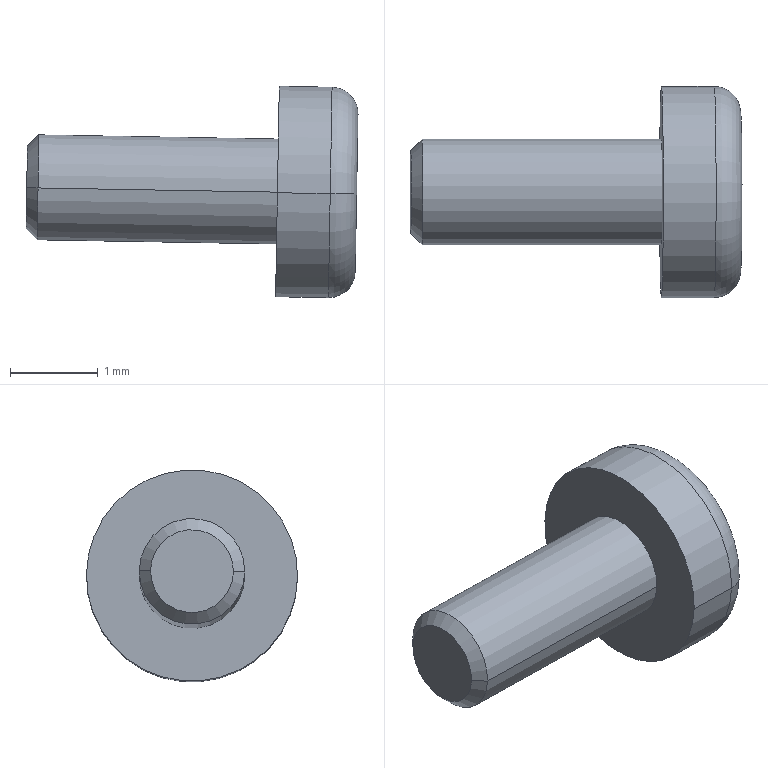Component | SolidWorks | 00-VacuumSuctionCupAssembly-1_06-M4PhillipsScrew-3 | 1 solid | 28 faces | box 3.77 x 2.4 x 2.41 mm | volume 7 mm3 | plane 16 | cylinder 8 | torus 2 | cone 2 | commonest cylinder face diameters 0.42 x4 1.2 x2 2.4 x2
STEP:
#1=CARTESIAN_POINT('',(2.87,5.778,1.592));
#2=VERTEX_POINT('',#1);
#3=CARTESIAN_POINT('',(2.87,5.873,1.594));
#4=VERTEX_POINT('',#3);
#5=CARTESIAN_POINT('',(2.87,5.826,1.593));
#6=DIRECTION('',(-0.9998,0.,0.01745));
#7=DIRECTION('',(0.0001976,0.9999,0.01132));
#8=AXIS2_PLACEMENT_3D('',#5,#6,#7);
#9=CIRCLE('',#8,0.04724);
#10=EDGE_CURVE('',#2,#4,#9,.T.);
#11=ORIENTED_EDGE('',*,*,#10,.F.);
#12=CARTESIAN_POINT('',(2.882,5.79,1.592));
#13=VERTEX_POINT('',#12);
#14=CARTESIAN_POINT('',(2.87,5.79,1.593));
#15=DIRECTION('',(0.01745,-0.01132,0.9998));
#16=DIRECTION('',(0.9998,0.,-0.01745));
#17=AXIS2_PLACEMENT_3D('',#14,#15,#16);
#18=CIRCLE('',#17,0.01181);
#19=EDGE_CURVE('',#2,#13,#18,.T.);
#20=ORIENTED_EDGE('',*,*,#19,.T.);
#21=CARTESIAN_POINT('',(2.882,5.861,1.593));
#22=VERTEX_POINT('',#21);
#23=CARTESIAN_POINT('',(2.882,5.826,1.593));
#24=DIRECTION('',(0.9998,-0.,-0.01745));
#25=DIRECTION('',(0.0001976,0.9999,0.01132));
#26=AXIS2_PLACEMENT_3D('',#23,#24,#25);
#27=CIRCLE('',#26,0.03543);
#28=EDGE_CURVE('',#22,#13,#27,.T.);
#29=ORIENTED_EDGE('',*,*,#28,.F.);
#30=CARTESIAN_POINT('',(2.87,5.861,1.593));
#31=DIRECTION('',(-0.01745,0.01132,-0.9998));
#32=DIRECTION('',(-0.9998,0.,0.01745));
#33=AXIS2_PLACEMENT_3D('',#30,#31,#32);
#34=CIRCLE('',#33,0.01181);
#35=EDGE_CURVE('',#4,#22,#34,.T.);
#36=ORIENTED_EDGE('',*,*,#35,.F.);
#37=EDGE_LOOP('',(#11,#20,#29,#36));
#38=FACE_OUTER_BOUND('',#37,.T.);
#39=CARTESIAN_POINT('',(2.87,5.826,1.593));
#40=DIRECTION('',(0.9998,-0.,-0.01745));
#41=DIRECTION('',(0.0001976,0.9999,0.01132));
#42=AXIS2_PLACEMENT_3D('',#39,#40,#41);
#43=TOROIDAL_SURFACE('',#42,0.03543,0.01181);
#44=ADVANCED_FACE('',(#38),#43,.T.);
#45=CARTESIAN_POINT('',(2.734,5.807,1.595));
#46=VERTEX_POINT('',#45);
#47=CARTESIAN_POINT('',(2.734,5.844,1.596));
#48=VERTEX_POINT('',#47);
#49=CARTESIAN_POINT('',(2.734,5.826,1.595));
#50=DIRECTION('',(-0.9998,0.,0.01745));
#51=DIRECTION('',(-0.0001976,-0.9999,-0.01132));
#52=AXIS2_PLACEMENT_3D('',#49,#50,#51);
#53=CIRCLE('',#52,0.01855);
#54=EDGE_CURVE('',#46,#48,#53,.T.);
#55=ORIENTED_EDGE('',*,*,#54,.F.);
#56=CARTESIAN_POINT('',(2.739,5.802,1.595));
#57=VERTEX_POINT('',#56);
#58=CARTESIAN_POINT('',(2.734,5.807,1.595));
#59=DIRECTION('',(0.7069,-0.7071,-0.02034));
#60=VECTOR('',#59,39.37);
#61=LINE('',#58,#60);
#62=EDGE_CURVE('',#46,#57,#61,.T.);
#63=ORIENTED_EDGE('',*,*,#62,.T.);
#64=CARTESIAN_POINT('',(2.739,5.849,1.596));
#65=VERTEX_POINT('',#64);
#66=CARTESIAN_POINT('',(2.739,5.826,1.595));
#67=DIRECTION('',(0.9998,-0.,-0.01745));
#68=DIRECTION('',(-0.0001976,-0.9999,-0.01132));
#69=AXIS2_PLACEMENT_3D('',#66,#67,#68);
#70=CIRCLE('',#69,0.02362);
#71=EDGE_CURVE('',#65,#57,#70,.T.);
#72=ORIENTED_EDGE('',*,*,#71,.F.);
#73=CARTESIAN_POINT('',(2.734,5.844,1.596));
#74=DIRECTION('',(0.7071,0.7071,-0.004337));
#75=VECTOR('',#74,39.37);
#76=LINE('',#73,#75);
#77=EDGE_CURVE('',#48,#65,#76,.T.);
#78=ORIENTED_EDGE('',*,*,#77,.F.);
#79=EDGE_LOOP('',(#55,#63,#72,#78));
#80=FACE_OUTER_BOUND('',#79,.T.);
#81=CARTESIAN_POINT('',(2.734,5.826,1.595));
#82=DIRECTION('',(0.9998,-0.,-0.01745));
#83=DIRECTION('',(0.0001976,0.9999,0.01132));
#84=AXIS2_PLACEMENT_3D('',#81,#82,#83);
#85=CONICAL_SURFACE('',#84,0.01855,0.7854);
#86=ADVANCED_FACE('',(#80),#85,.T.);
#87=ORIENTED_EDGE('',*,*,#71,.T.);
#88=CARTESIAN_POINT('',(2.846,5.802,1.593));
#89=VERTEX_POINT('',#88);
#90=CARTESIAN_POINT('',(2.734,5.802,1.595));
#91=DIRECTION('',(0.9998,-0.,-0.01745));
#92=VECTOR('',#91,39.37);
#93=LINE('',#90,#92);
#94=EDGE_CURVE('',#57,#89,#93,.T.);
#95=ORIENTED_EDGE('',*,*,#94,.T.);
#96=CARTESIAN_POINT('',(2.846,5.849,1.594));
#97=VERTEX_POINT('',#96);
#98=CARTESIAN_POINT('',(2.846,5.826,1.593));
#99=DIRECTION('',(-0.9998,0.,0.01745));
#100=DIRECTION('',(-0.0001976,-0.9999,-0.01132));
#101=AXIS2_PLACEMENT_3D('',#98,#99,#100);
#102=CIRCLE('',#101,0.02362);
#103=EDGE_CURVE('',#89,#97,#102,.T.);
#104=ORIENTED_EDGE('',*,*,#103,.T.);
#105=CARTESIAN_POINT('',(2.734,5.849,1.596));
#106=DIRECTION('',(0.9998,-0.,-0.01745));
#107=VECTOR('',#106,39.37);
#108=LINE('',#105,#107);
#109=EDGE_CURVE('',#65,#97,#108,.T.);
#110=ORIENTED_EDGE('',*,*,#109,.F.);
#111=EDGE_LOOP('',(#87,#95,#104,#110));
#112=FACE_OUTER_BOUND('',#111,.T.);
#113=CARTESIAN_POINT('',(2.734,5.826,1.595));
#114=DIRECTION('',(0.9998,-0.,-0.01745));
#115=DIRECTION('',(0.0001976,0.9999,0.01132));
#116=AXIS2_PLACEMENT_3D('',#113,#114,#115);
#117=CYLINDRICAL_SURFACE('',#116,0.02362);
#118=ADVANCED_FACE('',(#112),#117,.T.);
#119=ORIENTED_EDGE('',*,*,#10,.T.);
#120=CARTESIAN_POINT('',(2.846,5.873,1.594));
#121=VERTEX_POINT('',#120);
#122=CARTESIAN_POINT('',(2.882,5.873,1.593));
#123=DIRECTION('',(-0.9998,0.,0.01745));
#124=VECTOR('',#123,39.37);
#125=LINE('',#122,#124);
#126=EDGE_CURVE('',#4,#121,#125,.T.);
#127=ORIENTED_EDGE('',*,*,#126,.T.);
#128=CARTESIAN_POINT('',(2.846,5.778,1.593));
#129=VERTEX_POINT('',#128);
#130=CARTESIAN_POINT('',(2.846,5.826,1.593));
#131=DIRECTION('',(-0.9998,0.,0.01745));
#132=DIRECTION('',(-0.0001976,-0.9999,-0.01132));
#133=AXIS2_PLACEMENT_3D('',#130,#131,#132);
#134=CIRCLE('',#133,0.04724);
#135=EDGE_CURVE('',#129,#121,#134,.T.);
#136=ORIENTED_EDGE('',*,*,#135,.F.);
#137=CARTESIAN_POINT('',(2.882,5.778,1.592));
#138=DIRECTION('',(-0.9998,0.,0.01745));
#139=VECTOR('',#138,39.37);
#140=LINE('',#137,#139);
#141=EDGE_CURVE('',#2,#129,#140,.T.);
#142=ORIENTED_EDGE('',*,*,#141,.F.);
#143=EDGE_LOOP('',(#119,#127,#136,#142));
#144=FACE_OUTER_BOUND('',#143,.T.);
#145=CARTESIAN_POINT('',(2.882,5.826,1.593));
#146=DIRECTION('',(-0.9998,0.,0.01745));
#147=DIRECTION('',(-0.0001976,-0.9999,-0.01132));
#148=AXIS2_PLACEMENT_3D('',#145,#146,#147);
#149=CYLINDRICAL_SURFACE('',#148,0.04724);
#150=ADVANCED_FACE('',(#144),#149,.T.);
#151=ORIENTED_EDGE('',*,*,#135,.T.);
#152=CARTESIAN_POINT('',(2.846,5.826,1.593));
#153=DIRECTION('',(-0.9998,0.,0.01745));
#154=DIRECTION('',(-0.0001976,-0.9999,-0.01132));
#155=AXIS2_PLACEMENT_3D('',#152,#153,#154);
#156=CIRCLE('',#155,0.04724);
#157=EDGE_CURVE('',#121,#129,#156,.T.);
#158=ORIENTED_EDGE('',*,*,#157,.T.);
#159=EDGE_LOOP('',(#151,#158));
#160=FACE_OUTER_BOUND('',#159,.T.);
#161=CARTESIAN_POINT('',(2.846,5.826,1.593));
#162=DIRECTION('',(-0.9998,0.,0.01745));
#163=DIRECTION('',(-0.0001976,-0.9999,-0.01132));
#164=AXIS2_PLACEMENT_3D('',#161,#162,#163);
#165=CIRCLE('',#164,0.02362);
#166=EDGE_CURVE('',#97,#89,#165,.T.);
#167=ORIENTED_EDGE('',*,*,#166,.F.);
#168=ORIENTED_EDGE('',*,*,#103,.F.);
#169=EDGE_LOOP('',(#167,#168));
#170=FACE_BOUND('',#169,.T.);
#171=CARTESIAN_POINT('',(2.846,5.826,1.593));
#172=DIRECTION('',(-0.9998,0.,0.01745));
#173=DIRECTION('',(-0.0001976,-0.9999,-0.01132));
#174=AXIS2_PLACEMENT_3D('',#171,#172,#173);
#175=PLANE('',#174);
#176=ADVANCED_FACE('',(#160,#170),#175,.T.);
#177=ORIENTED_EDGE('',*,*,#126,.F.);
#178=CARTESIAN_POINT('',(2.87,5.826,1.593));
#179=DIRECTION('',(-0.9998,0.,0.01745));
#180=DIRECTION('',(0.0001976,0.9999,0.01132));
#181=AXIS2_PLACEMENT_3D('',#178,#179,#180);
#182=CIRCLE('',#181,0.04724);
#183=EDGE_CURVE('',#4,#2,#182,.T.);
#184=ORIENTED_EDGE('',*,*,#183,.T.);
#185=ORIENTED_EDGE('',*,*,#141,.T.);
#186=ORIENTED_EDGE('',*,*,#157,.F.);
#187=EDGE_LOOP('',(#177,#184,#185,#186));
#188=FACE_OUTER_BOUND('',#187,.T.);
#189=CARTESIAN_POINT('',(2.882,5.826,1.593));
#190=DIRECTION('',(-0.9998,0.,0.01745));
#191=DIRECTION('',(-0.0001976,-0.9999,-0.01132));
#192=AXIS2_PLACEMENT_3D('',#189,#190,#191);
#193=CYLINDRICAL_SURFACE('',#192,0.04724);
#194=ADVANCED_FACE('',(#188),#193,.T.);
#195=ORIENTED_EDGE('',*,*,#28,.T.);
#196=CARTESIAN_POINT('',(2.882,5.826,1.593));
#197=DIRECTION('',(0.9998,-0.,-0.01745));
#198=DIRECTION('',(0.0001976,0.9999,0.01132));
#199=AXIS2_PLACEMENT_3D('',#196,#197,#198);
#200=CIRCLE('',#199,0.03543);
#201=EDGE_CURVE('',#13,#22,#200,.T.);
#202=ORIENTED_EDGE('',*,*,#201,.T.);
#203=EDGE_LOOP('',(#195,#202));
#204=FACE_OUTER_BOUND('',#203,.T.);
#205=CARTESIAN_POINT('',(2.882,5.811,1.599));
#206=VERTEX_POINT('',#205);
#207=CARTESIAN_POINT('',(2.882,5.8,1.598));
#208=VERTEX_POINT('',#207);
#209=CARTESIAN_POINT('',(2.882,5.82,1.599));
#210=DIRECTION('',(-0.0001976,-0.9999,-0.01132));
#211=VECTOR('',#210,39.37);
#212=LINE('',#209,#211);
#213=EDGE_CURVE('',#206,#208,#212,.T.);
#214=ORIENTED_EDGE('',*,*,#213,.F.);
#215=CARTESIAN_POINT('',(2.882,5.82,1.607));
#216=VERTEX_POINT('',#215);
#217=CARTESIAN_POINT('',(2.882,5.811,1.607));
#218=DIRECTION('',(0.9998,-0.,-0.01745));
#219=DIRECTION('',(0.0001976,0.9999,0.01132));
#220=AXIS2_PLACEMENT_3D('',#217,#218,#219);
#221=CIRCLE('',#220,0.008268);
#222=EDGE_CURVE('',#206,#216,#221,.T.);
#223=ORIENTED_EDGE('',*,*,#222,.T.);
#224=CARTESIAN_POINT('',(2.882,5.819,1.619));
#225=VERTEX_POINT('',#224);
#226=CARTESIAN_POINT('',(2.882,5.819,1.619));
#227=DIRECTION('',(-0.01745,0.01132,-0.9998));
#228=VECTOR('',#227,39.37);
#229=LINE('',#226,#228);
#230=EDGE_CURVE('',#225,#216,#229,.T.);
#231=ORIENTED_EDGE('',*,*,#230,.F.);
#232=CARTESIAN_POINT('',(2.882,5.831,1.619));
#233=VERTEX_POINT('',#232);
#234=CARTESIAN_POINT('',(2.882,5.831,1.619));
#235=DIRECTION('',(-0.0001976,-0.9999,-0.01132));
#236=VECTOR('',#235,39.37);
#237=LINE('',#234,#236);
#238=EDGE_CURVE('',#233,#225,#237,.T.);
#239=ORIENTED_EDGE('',*,*,#238,.F.);
#240=CARTESIAN_POINT('',(2.882,5.831,1.607));
#241=VERTEX_POINT('',#240);
#242=CARTESIAN_POINT('',(2.882,5.832,1.599));
#243=DIRECTION('',(0.01745,-0.01132,0.9998));
#244=VECTOR('',#243,39.37);
#245=LINE('',#242,#244);
#246=EDGE_CURVE('',#241,#233,#245,.T.);
#247=ORIENTED_EDGE('',*,*,#246,.F.);
#248=CARTESIAN_POINT('',(2.882,5.84,1.599));
#249=VERTEX_POINT('',#248);
#250=CARTESIAN_POINT('',(2.882,5.84,1.607));
#251=DIRECTION('',(0.9998,-0.,-0.01745));
#252=DIRECTION('',(0.0001976,0.9999,0.01132));
#253=AXIS2_PLACEMENT_3D('',#250,#251,#252);
#254=CIRCLE('',#253,0.008268);
#255=EDGE_CURVE('',#241,#249,#254,.T.);
#256=ORIENTED_EDGE('',*,*,#255,.T.);
#257=CARTESIAN_POINT('',(2.882,5.852,1.599));
#258=VERTEX_POINT('',#257);
#259=CARTESIAN_POINT('',(2.882,5.852,1.599));
#260=DIRECTION('',(-0.0001976,-0.9999,-0.01132));
#261=VECTOR('',#260,39.37);
#262=LINE('',#259,#261);
#263=EDGE_CURVE('',#258,#249,#262,.T.);
#264=ORIENTED_EDGE('',*,*,#263,.F.);
#265=CARTESIAN_POINT('',(2.882,5.852,1.587));
#266=VERTEX_POINT('',#265);
#267=CARTESIAN_POINT('',(2.882,5.852,1.587));
#268=DIRECTION('',(0.01745,-0.01132,0.9998));
#269=VECTOR('',#268,39.37);
#270=LINE('',#267,#269);
#271=EDGE_CURVE('',#266,#258,#270,.T.);
#272=ORIENTED_EDGE('',*,*,#271,.F.);
#273=CARTESIAN_POINT('',(2.882,5.84,1.587));
#274=VERTEX_POINT('',#273);
#275=CARTESIAN_POINT('',(2.882,5.832,1.587));
#276=DIRECTION('',(0.0001976,0.9999,0.01132));
#277=VECTOR('',#276,39.37);
#278=LINE('',#275,#277);
#279=EDGE_CURVE('',#274,#266,#278,.T.);
#280=ORIENTED_EDGE('',*,*,#279,.F.);
#281=CARTESIAN_POINT('',(2.882,5.832,1.579));
#282=VERTEX_POINT('',#281);
#283=CARTESIAN_POINT('',(2.882,5.84,1.579));
#284=DIRECTION('',(0.9998,-0.,-0.01745));
#285=DIRECTION('',(0.0001976,0.9999,0.01132));
#286=AXIS2_PLACEMENT_3D('',#283,#284,#285);
#287=CIRCLE('',#286,0.008268);
#288=EDGE_CURVE('',#274,#282,#287,.T.);
#289=ORIENTED_EDGE('',*,*,#288,.T.);
#290=CARTESIAN_POINT('',(2.881,5.832,1.567));
#291=VERTEX_POINT('',#290);
#292=CARTESIAN_POINT('',(2.881,5.832,1.567));
#293=DIRECTION('',(0.01745,-0.01132,0.9998));
#294=VECTOR('',#293,39.37);
#295=LINE('',#292,#294);
#296=EDGE_CURVE('',#291,#282,#295,.T.);
#297=ORIENTED_EDGE('',*,*,#296,.F.);
#298=CARTESIAN_POINT('',(2.881,5.82,1.567));
#299=VERTEX_POINT('',#298);
#300=CARTESIAN_POINT('',(2.881,5.82,1.567));
#301=DIRECTION('',(0.0001976,0.9999,0.01132));
#302=VECTOR('',#301,39.37);
#303=LINE('',#300,#302);
#304=EDGE_CURVE('',#299,#291,#303,.T.);
#305=ORIENTED_EDGE('',*,*,#304,.F.);
#306=CARTESIAN_POINT('',(2.882,5.82,1.579));
#307=VERTEX_POINT('',#306);
#308=CARTESIAN_POINT('',(2.882,5.82,1.587));
#309=DIRECTION('',(-0.01745,0.01132,-0.9998));
#310=VECTOR('',#309,39.37);
#311=LINE('',#308,#310);
#312=EDGE_CURVE('',#307,#299,#311,.T.);
#313=ORIENTED_EDGE('',*,*,#312,.F.);
#314=CARTESIAN_POINT('',(2.882,5.812,1.587));
#315=VERTEX_POINT('',#314);
#316=CARTESIAN_POINT('',(2.882,5.812,1.578));
#317=DIRECTION('',(0.9998,-0.,-0.01745));
#318=DIRECTION('',(0.0001976,0.9999,0.01132));
#319=AXIS2_PLACEMENT_3D('',#316,#317,#318);
#320=CIRCLE('',#319,0.008268);
#321=EDGE_CURVE('',#307,#315,#320,.T.);
#322=ORIENTED_EDGE('',*,*,#321,.T.);
#323=CARTESIAN_POINT('',(2.882,5.8,1.587));
#324=VERTEX_POINT('',#323);
#325=CARTESIAN_POINT('',(2.882,5.8,1.587));
#326=DIRECTION('',(0.0001976,0.9999,0.01132));
#327=VECTOR('',#326,39.37);
#328=LINE('',#325,#327);
#329=EDGE_CURVE('',#324,#315,#328,.T.);
#330=ORIENTED_EDGE('',*,*,#329,.F.);
#331=CARTESIAN_POINT('',(2.882,5.8,1.598));
#332=DIRECTION('',(-0.01745,0.01132,-0.9998));
#333=VECTOR('',#332,39.37);
#334=LINE('',#331,#333);
#335=EDGE_CURVE('',#208,#324,#334,.T.);
#336=ORIENTED_EDGE('',*,*,#335,.F.);
#337=EDGE_LOOP('',(#214,#223,#231,#239,#247,#256,#264,#272,#280,#289,#297,#305,#313,#322,#330,#336));
#338=FACE_BOUND('',#337,.T.);
#339=CARTESIAN_POINT('',(2.883,5.825,1.64));
#340=DIRECTION('',(0.9998,-0.,-0.01745));
#341=DIRECTION('',(0.0001976,0.9999,0.01132));
#342=AXIS2_PLACEMENT_3D('',#339,#340,#341);
#343=PLANE('',#342);
#344=ADVANCED_FACE('',(#204,#338),#343,.T.);
#345=ORIENTED_EDGE('',*,*,#94,.F.);
#346=CARTESIAN_POINT('',(2.739,5.826,1.595));
#347=DIRECTION('',(0.9998,-0.,-0.01745));
#348=DIRECTION('',(-0.0001976,-0.9999,-0.01132));
#349=AXIS2_PLACEMENT_3D('',#346,#347,#348);
#350=CIRCLE('',#349,0.02362);
#351=EDGE_CURVE('',#57,#65,#350,.T.);
#352=ORIENTED_EDGE('',*,*,#351,.T.);
#353=ORIENTED_EDGE('',*,*,#109,.T.);
#354=ORIENTED_EDGE('',*,*,#166,.T.);
#355=EDGE_LOOP('',(#345,#352,#353,#354));
#356=FACE_OUTER_BOUND('',#355,.T.);
#357=CARTESIAN_POINT('',(2.734,5.826,1.595));
#358=DIRECTION('',(0.9998,-0.,-0.01745));
#359=DIRECTION('',(0.0001976,0.9999,0.01132));
#360=AXIS2_PLACEMENT_3D('',#357,#358,#359);
#361=CYLINDRICAL_SURFACE('',#360,0.02362);
#362=ADVANCED_FACE('',(#356),#361,.T.);
#363=CARTESIAN_POINT('',(2.734,5.826,1.595));
#364=DIRECTION('',(-0.9998,0.,0.01745));
#365=DIRECTION('',(-0.0001976,-0.9999,-0.01132));
#366=AXIS2_PLACEMENT_3D('',#363,#364,#365);
#367=CIRCLE('',#366,0.01855);
#368=EDGE_CURVE('',#48,#46,#367,.T.);
#369=ORIENTED_EDGE('',*,*,#368,.T.);
#370=ORIENTED_EDGE('',*,*,#54,.T.);
#371=EDGE_LOOP('',(#369,#370));
#372=FACE_OUTER_BOUND('',#371,.T.);
#373=CARTESIAN_POINT('',(2.734,5.826,1.595));
#374=DIRECTION('',(-0.9998,0.,0.01745));
#375=DIRECTION('',(-0.0001976,-0.9999,-0.01132));
#376=AXIS2_PLACEMENT_3D('',#373,#374,#375);
#377=PLANE('',#376);
#378=ADVANCED_FACE('',(#372),#377,.T.);
#379=CARTESIAN_POINT('',(2.858,5.84,1.587));
#380=VERTEX_POINT('',#379);
#381=CARTESIAN_POINT('',(2.858,5.852,1.588));
#382=VERTEX_POINT('',#381);
#383=CARTESIAN_POINT('',(2.858,5.832,1.587));
#384=DIRECTION('',(0.0001976,0.9999,0.01132));
#385=VECTOR('',#384,39.37);
#386=LINE('',#383,#385);
#387=EDGE_CURVE('',#380,#382,#386,.T.);
#388=ORIENTED_EDGE('',*,*,#387,.F.);
#389=CARTESIAN_POINT('',(2.858,5.84,1.587));
#390=DIRECTION('',(0.9998,-0.,-0.01745));
#391=VECTOR('',#390,39.37);
#392=LINE('',#389,#391);
#393=EDGE_CURVE('',#380,#274,#392,.T.);
#394=ORIENTED_EDGE('',*,*,#393,.T.);
#395=ORIENTED_EDGE('',*,*,#279,.T.);
#396=CARTESIAN_POINT('',(2.858,5.852,1.588));
#397=DIRECTION('',(0.9998,-0.,-0.01745));
#398=VECTOR('',#397,39.37);
#399=LINE('',#396,#398);
#400=EDGE_CURVE('',#382,#266,#399,.T.);
#401=ORIENTED_EDGE('',*,*,#400,.F.);
#402=EDGE_LOOP('',(#388,#394,#395,#401));
#403=FACE_OUTER_BOUND('',#402,.T.);
#404=CARTESIAN_POINT('',(2.858,5.832,1.587));
#405=DIRECTION('',(-0.01745,0.01132,-0.9998));
#406=DIRECTION('',(-0.0001976,-0.9999,-0.01132));
#407=AXIS2_PLACEMENT_3D('',#404,#405,#406);
#408=PLANE('',#407);
#409=ADVANCED_FACE('',(#403),#408,.F.);
#410=ORIENTED_EDGE('',*,*,#296,.T.);
#411=CARTESIAN_POINT('',(2.858,5.832,1.579));
#412=VERTEX_POINT('',#411);
#413=CARTESIAN_POINT('',(2.858,5.832,1.579));
#414=DIRECTION('',(-0.9998,0.,0.01745));
#415=VECTOR('',#414,39.37);
#416=LINE('',#413,#415);
#417=EDGE_CURVE('',#282,#412,#416,.T.);
#418=ORIENTED_EDGE('',*,*,#417,.T.);
#419=CARTESIAN_POINT('',(2.858,5.832,1.567));
#420=VERTEX_POINT('',#419);
#421=CARTESIAN_POINT('',(2.858,5.832,1.567));
#422=DIRECTION('',(0.01745,-0.01132,0.9998));
#423=VECTOR('',#422,39.37);
#424=LINE('',#421,#423);
#425=EDGE_CURVE('',#420,#412,#424,.T.);
#426=ORIENTED_EDGE('',*,*,#425,.F.);
#427=CARTESIAN_POINT('',(2.858,5.832,1.567));
#428=DIRECTION('',(0.9998,-0.,-0.01745));
#429=VECTOR('',#428,39.37);
#430=LINE('',#427,#429);
#431=EDGE_CURVE('',#420,#291,#430,.T.);
#432=ORIENTED_EDGE('',*,*,#431,.T.);
#433=EDGE_LOOP('',(#410,#418,#426,#432));
#434=FACE_OUTER_BOUND('',#433,.T.);
#435=CARTESIAN_POINT('',(2.858,5.832,1.567));
#436=DIRECTION('',(0.0001976,0.9999,0.01132));
#437=DIRECTION('',(-0.9998,0.,0.01745));
#438=AXIS2_PLACEMENT_3D('',#435,#436,#437);
#439=PLANE('',#438);
#440=ADVANCED_FACE('',(#434),#439,.F.);
#441=ORIENTED_EDGE('',*,*,#304,.T.);
#442=ORIENTED_EDGE('',*,*,#431,.F.);
#443=CARTESIAN_POINT('',(2.858,5.82,1.567));
#444=VERTEX_POINT('',#443);
#445=CARTESIAN_POINT('',(2.858,5.82,1.567));
#446=DIRECTION('',(0.0001976,0.9999,0.01132));
#447=VECTOR('',#446,39.37);
#448=LINE('',#445,#447);
#449=EDGE_CURVE('',#444,#420,#448,.T.);
#450=ORIENTED_EDGE('',*,*,#449,.F.);
#451=CARTESIAN_POINT('',(2.858,5.82,1.567));
#452=DIRECTION('',(0.9998,-0.,-0.01745));
#453=VECTOR('',#452,39.37);
#454=LINE('',#451,#453);
#455=EDGE_CURVE('',#444,#299,#454,.T.);
#456=ORIENTED_EDGE('',*,*,#455,.T.);
#457=EDGE_LOOP('',(#441,#442,#450,#456));
#458=FACE_OUTER_BOUND('',#457,.T.);
#459=CARTESIAN_POINT('',(2.858,5.82,1.567));
#460=DIRECTION('',(-0.01745,0.01132,-0.9998));
#461=DIRECTION('',(-0.0001976,-0.9999,-0.01132));
#462=AXIS2_PLACEMENT_3D('',#459,#460,#461);
#463=PLANE('',#462);
#464=ADVANCED_FACE('',(#458),#463,.F.);
#465=CARTESIAN_POINT('',(2.858,5.82,1.579));
#466=VERTEX_POINT('',#465);
#467=CARTESIAN_POINT('',(2.858,5.82,1.587));
#468=DIRECTION('',(-0.01745,0.01132,-0.9998));
#469=VECTOR('',#468,39.37);
#470=LINE('',#467,#469);
#471=EDGE_CURVE('',#466,#444,#470,.T.);
#472=ORIENTED_EDGE('',*,*,#471,.F.);
#473=CARTESIAN_POINT('',(2.858,5.82,1.579));
#474=DIRECTION('',(0.9998,-0.,-0.01745));
#475=VECTOR('',#474,39.37);
#476=LINE('',#473,#475);
#477=EDGE_CURVE('',#466,#307,#476,.T.);
#478=ORIENTED_EDGE('',*,*,#477,.T.);
#479=ORIENTED_EDGE('',*,*,#312,.T.);
#480=ORIENTED_EDGE('',*,*,#455,.F.);
#481=EDGE_LOOP('',(#472,#478,#479,#480));
#482=FACE_OUTER_BOUND('',#481,.T.);
#483=CARTESIAN_POINT('',(2.858,5.82,1.587));
#484=DIRECTION('',(-0.0001976,-0.9999,-0.01132));
#485=DIRECTION('',(0.9998,-0.,-0.01745));
#486=AXIS2_PLACEMENT_3D('',#483,#484,#485);
#487=PLANE('',#486);
#488=ADVANCED_FACE('',(#482),#487,.F.);
#489=ORIENTED_EDGE('',*,*,#329,.T.);
#490=CARTESIAN_POINT('',(2.858,5.812,1.587));
#491=VERTEX_POINT('',#490);
#492=CARTESIAN_POINT('',(2.858,5.812,1.587));
#493=DIRECTION('',(-0.9998,0.,0.01745));
#494=VECTOR('',#493,39.37);
#495=LINE('',#492,#494);
#496=EDGE_CURVE('',#315,#491,#495,.T.);
#497=ORIENTED_EDGE('',*,*,#496,.T.);
#498=CARTESIAN_POINT('',(2.858,5.8,1.587));
#499=VERTEX_POINT('',#498);
#500=CARTESIAN_POINT('',(2.858,5.8,1.587));
#501=DIRECTION('',(0.0001976,0.9999,0.01132));
#502=VECTOR('',#501,39.37);
#503=LINE('',#500,#502);
#504=EDGE_CURVE('',#499,#491,#503,.T.);
#505=ORIENTED_EDGE('',*,*,#504,.F.);
#506=CARTESIAN_POINT('',(2.858,5.8,1.587));
#507=DIRECTION('',(0.9998,-0.,-0.01745));
#508=VECTOR('',#507,39.37);
#509=LINE('',#506,#508);
#510=EDGE_CURVE('',#499,#324,#509,.T.);
#511=ORIENTED_EDGE('',*,*,#510,.T.);
#512=EDGE_LOOP('',(#489,#497,#505,#511));
#513=FACE_OUTER_BOUND('',#512,.T.);
#514=CARTESIAN_POINT('',(2.858,5.8,1.587));
#515=DIRECTION('',(-0.01745,0.01132,-0.9998));
#516=DIRECTION('',(-0.0001976,-0.9999,-0.01132));
#517=AXIS2_PLACEMENT_3D('',#514,#515,#516);
#518=PLANE('',#517);
#519=ADVANCED_FACE('',(#513),#518,.F.);
#520=ORIENTED_EDGE('',*,*,#335,.T.);
#521=ORIENTED_EDGE('',*,*,#510,.F.);
#522=CARTESIAN_POINT('',(2.858,5.8,1.599));
#523=VERTEX_POINT('',#522);
#524=CARTESIAN_POINT('',(2.858,5.8,1.599));
#525=DIRECTION('',(-0.01745,0.01132,-0.9998));
#526=VECTOR('',#525,39.37);
#527=LINE('',#524,#526);
#528=EDGE_CURVE('',#523,#499,#527,.T.);
#529=ORIENTED_EDGE('',*,*,#528,.F.);
#530=CARTESIAN_POINT('',(2.858,5.8,1.599));
#531=DIRECTION('',(0.9998,-0.,-0.01745));
#532=VECTOR('',#531,39.37);
#533=LINE('',#530,#532);
#534=EDGE_CURVE('',#523,#208,#533,.T.);
#535=ORIENTED_EDGE('',*,*,#534,.T.);
#536=EDGE_LOOP('',(#520,#521,#529,#535));
#537=FACE_OUTER_BOUND('',#536,.T.);
#538=CARTESIAN_POINT('',(2.858,5.8,1.599));
#539=DIRECTION('',(-0.0001976,-0.9999,-0.01132));
#540=DIRECTION('',(0.9998,-0.,-0.01745));
#541=AXIS2_PLACEMENT_3D('',#538,#539,#540);
#542=PLANE('',#541);
#543=ADVANCED_FACE('',(#537),#542,.F.);
#544=CARTESIAN_POINT('',(2.858,5.811,1.599));
#545=VERTEX_POINT('',#544);
#546=CARTESIAN_POINT('',(2.858,5.82,1.599));
#547=DIRECTION('',(-0.0001976,-0.9999,-0.01132));
#548=VECTOR('',#547,39.37);
#549=LINE('',#546,#548);
#550=EDGE_CURVE('',#545,#523,#549,.T.);
#551=ORIENTED_EDGE('',*,*,#550,.F.);
#552=CARTESIAN_POINT('',(2.858,5.811,1.599));
#553=DIRECTION('',(0.9998,-0.,-0.01745));
#554=VECTOR('',#553,39.37);
#555=LINE('',#552,#554);
#556=EDGE_CURVE('',#545,#206,#555,.T.);
#557=ORIENTED_EDGE('',*,*,#556,.T.);
#558=ORIENTED_EDGE('',*,*,#213,.T.);
#559=ORIENTED_EDGE('',*,*,#534,.F.);
#560=EDGE_LOOP('',(#551,#557,#558,#559));
#561=FACE_OUTER_BOUND('',#560,.T.);
#562=CARTESIAN_POINT('',(2.858,5.82,1.599));
#563=DIRECTION('',(0.01745,-0.01132,0.9998));
#564=DIRECTION('',(0.0001976,0.9999,0.01132));
#565=AXIS2_PLACEMENT_3D('',#562,#563,#564);
#566=PLANE('',#565);
#567=ADVANCED_FACE('',(#561),#566,.F.);
#568=ORIENTED_EDGE('',*,*,#230,.T.);
#569=CARTESIAN_POINT('',(2.858,5.82,1.607));
#570=VERTEX_POINT('',#569);
#571=CARTESIAN_POINT('',(2.858,5.82,1.607));
#572=DIRECTION('',(-0.9998,0.,0.01745));
#573=VECTOR('',#572,39.37);
#574=LINE('',#571,#573);
#575=EDGE_CURVE('',#216,#570,#574,.T.);
#576=ORIENTED_EDGE('',*,*,#575,.T.);
#577=CARTESIAN_POINT('',(2.859,5.819,1.619));
#578=VERTEX_POINT('',#577);
#579=CARTESIAN_POINT('',(2.859,5.819,1.619));
#580=DIRECTION('',(-0.01745,0.01132,-0.9998));
#581=VECTOR('',#580,39.37);
#582=LINE('',#579,#581);
#583=EDGE_CURVE('',#578,#570,#582,.T.);
#584=ORIENTED_EDGE('',*,*,#583,.F.);
#585=CARTESIAN_POINT('',(2.859,5.819,1.619));
#586=DIRECTION('',(0.9998,-0.,-0.01745));
#587=VECTOR('',#586,39.37);
#588=LINE('',#585,#587);
#589=EDGE_CURVE('',#578,#225,#588,.T.);
#590=ORIENTED_EDGE('',*,*,#589,.T.);
#591=EDGE_LOOP('',(#568,#576,#584,#590));
#592=FACE_OUTER_BOUND('',#591,.T.);
#593=CARTESIAN_POINT('',(2.859,5.819,1.619));
#594=DIRECTION('',(-0.0001976,-0.9999,-0.01132));
#595=DIRECTION('',(0.9998,-0.,-0.01745));
#596=AXIS2_PLACEMENT_3D('',#593,#594,#595);
#597=PLANE('',#596);
#598=ADVANCED_FACE('',(#592),#597,.F.);
#599=ORIENTED_EDGE('',*,*,#238,.T.);
#600=ORIENTED_EDGE('',*,*,#589,.F.);
#601=CARTESIAN_POINT('',(2.859,5.831,1.619));
#602=VERTEX_POINT('',#601);
#603=CARTESIAN_POINT('',(2.859,5.831,1.619));
#604=DIRECTION('',(-0.0001976,-0.9999,-0.01132));
#605=VECTOR('',#604,39.37);
#606=LINE('',#603,#605);
#607=EDGE_CURVE('',#602,#578,#606,.T.);
#608=ORIENTED_EDGE('',*,*,#607,.F.);
#609=CARTESIAN_POINT('',(2.859,5.831,1.619));
#610=DIRECTION('',(0.9998,-0.,-0.01745));
#611=VECTOR('',#610,39.37);
#612=LINE('',#609,#611);
#613=EDGE_CURVE('',#602,#233,#612,.T.);
#614=ORIENTED_EDGE('',*,*,#613,.T.);
#615=EDGE_LOOP('',(#599,#600,#608,#614));
#616=FACE_OUTER_BOUND('',#615,.T.);
#617=CARTESIAN_POINT('',(2.859,5.831,1.619));
#618=DIRECTION('',(0.01745,-0.01132,0.9998));
#619=DIRECTION('',(0.0001976,0.9999,0.01132));
#620=AXIS2_PLACEMENT_3D('',#617,#618,#619);
#621=PLANE('',#620);
#622=ADVANCED_FACE('',(#616),#621,.F.);
#623=CARTESIAN_POINT('',(2.858,5.831,1.607));
#624=VERTEX_POINT('',#623);
#625=CARTESIAN_POINT('',(2.858,5.832,1.599));
#626=DIRECTION('',(0.01745,-0.01132,0.9998));
#627=VECTOR('',#626,39.37);
#628=LINE('',#625,#627);
#629=EDGE_CURVE('',#624,#602,#628,.T.);
#630=ORIENTED_EDGE('',*,*,#629,.F.);
#631=CARTESIAN_POINT('',(2.858,5.831,1.607));
#632=DIRECTION('',(0.9998,-0.,-0.01745));
#633=VECTOR('',#632,39.37);
#634=LINE('',#631,#633);
#635=EDGE_CURVE('',#624,#241,#634,.T.);
#636=ORIENTED_EDGE('',*,*,#635,.T.);
#637=ORIENTED_EDGE('',*,*,#246,.T.);
#638=ORIENTED_EDGE('',*,*,#613,.F.);
#639=EDGE_LOOP('',(#630,#636,#637,#638));
#640=FACE_OUTER_BOUND('',#639,.T.);
#641=CARTESIAN_POINT('',(2.858,5.832,1.599));
#642=DIRECTION('',(0.0001976,0.9999,0.01132));
#643=DIRECTION('',(-0.9998,0.,0.01745));
#644=AXIS2_PLACEMENT_3D('',#641,#642,#643);
#645=PLANE('',#644);
#646=ADVANCED_FACE('',(#640),#645,.F.);
#647=ORIENTED_EDGE('',*,*,#263,.T.);
#648=CARTESIAN_POINT('',(2.858,5.84,1.599));
#649=VERTEX_POINT('',#648);
#650=CARTESIAN_POINT('',(2.858,5.84,1.599));
#651=DIRECTION('',(-0.9998,0.,0.01745));
#652=VECTOR('',#651,39.37);
#653=LINE('',#650,#652);
#654=EDGE_CURVE('',#249,#649,#653,.T.);
#655=ORIENTED_EDGE('',*,*,#654,.T.);
#656=CARTESIAN_POINT('',(2.858,5.852,1.599));
#657=VERTEX_POINT('',#656);
#658=CARTESIAN_POINT('',(2.858,5.852,1.599));
#659=DIRECTION('',(-0.0001976,-0.9999,-0.01132));
#660=VECTOR('',#659,39.37);
#661=LINE('',#658,#660);
#662=EDGE_CURVE('',#657,#649,#661,.T.);
#663=ORIENTED_EDGE('',*,*,#662,.F.);
#664=CARTESIAN_POINT('',(2.858,5.852,1.599));
#665=DIRECTION('',(0.9998,-0.,-0.01745));
#666=VECTOR('',#665,39.37);
#667=LINE('',#664,#666);
#668=EDGE_CURVE('',#657,#258,#667,.T.);
#669=ORIENTED_EDGE('',*,*,#668,.T.);
#670=EDGE_LOOP('',(#647,#655,#663,#669));
#671=FACE_OUTER_BOUND('',#670,.T.);
#672=CARTESIAN_POINT('',(2.858,5.852,1.599));
#673=DIRECTION('',(0.01745,-0.01132,0.9998));
#674=DIRECTION('',(0.0001976,0.9999,0.01132));
#675=AXIS2_PLACEMENT_3D('',#672,#673,#674);
#676=PLANE('',#675);
#677=ADVANCED_FACE('',(#671),#676,.F.);
#678=ORIENTED_EDGE('',*,*,#271,.T.);
#679=ORIENTED_EDGE('',*,*,#668,.F.);
#680=CARTESIAN_POINT('',(2.858,5.852,1.588));
#681=DIRECTION('',(0.01745,-0.01132,0.9998));
#682=VECTOR('',#681,39.37);
#683=LINE('',#680,#682);
#684=EDGE_CURVE('',#382,#657,#683,.T.);
#685=ORIENTED_EDGE('',*,*,#684,.F.);
#686=ORIENTED_EDGE('',*,*,#400,.T.);
#687=EDGE_LOOP('',(#678,#679,#685,#686));
#688=FACE_OUTER_BOUND('',#687,.T.);
#689=CARTESIAN_POINT('',(2.858,5.852,1.588));
#690=DIRECTION('',(0.0001976,0.9999,0.01132));
#691=DIRECTION('',(-0.9998,0.,0.01745));
#692=AXIS2_PLACEMENT_3D('',#689,#690,#691);
#693=PLANE('',#692);
#694=ADVANCED_FACE('',(#688),#693,.F.);
#695=ORIENTED_EDGE('',*,*,#425,.T.);
#696=CARTESIAN_POINT('',(2.858,5.84,1.579));
#697=DIRECTION('',(-0.9998,0.,0.01745));
#698=DIRECTION('',(0.0001976,0.9999,0.01132));
#699=AXIS2_PLACEMENT_3D('',#696,#697,#698);
#700=CIRCLE('',#699,0.008268);
#701=EDGE_CURVE('',#412,#380,#700,.T.);
#702=ORIENTED_EDGE('',*,*,#701,.T.);
#703=ORIENTED_EDGE('',*,*,#387,.T.);
#704=ORIENTED_EDGE('',*,*,#684,.T.);
#705=ORIENTED_EDGE('',*,*,#662,.T.);
#706=CARTESIAN_POINT('',(2.858,5.84,1.608));
#707=DIRECTION('',(-0.9998,0.,0.01745));
#708=DIRECTION('',(0.0001976,0.9999,0.01132));
#709=AXIS2_PLACEMENT_3D('',#706,#707,#708);
#710=CIRCLE('',#709,0.008268);
#711=EDGE_CURVE('',#649,#624,#710,.T.);
#712=ORIENTED_EDGE('',*,*,#711,.T.);
#713=ORIENTED_EDGE('',*,*,#629,.T.);
#714=ORIENTED_EDGE('',*,*,#607,.T.);
#715=ORIENTED_EDGE('',*,*,#583,.T.);
#716=CARTESIAN_POINT('',(2.858,5.811,1.607));
#717=DIRECTION('',(-0.9998,0.,0.01745));
#718=DIRECTION('',(0.0001976,0.9999,0.01132));
#719=AXIS2_PLACEMENT_3D('',#716,#717,#718);
#720=CIRCLE('',#719,0.008268);
#721=EDGE_CURVE('',#570,#545,#720,.T.);
#722=ORIENTED_EDGE('',*,*,#721,.T.);
#723=ORIENTED_EDGE('',*,*,#550,.T.);
#724=ORIENTED_EDGE('',*,*,#528,.T.);
#725=ORIENTED_EDGE('',*,*,#504,.T.);
#726=CARTESIAN_POINT('',(2.858,5.812,1.579));
#727=DIRECTION('',(-0.9998,0.,0.01745));
#728=DIRECTION('',(0.0001976,0.9999,0.01132));
#729=AXIS2_PLACEMENT_3D('',#726,#727,#728);
#730=CIRCLE('',#729,0.008268);
#731=EDGE_CURVE('',#491,#466,#730,.T.);
#732=ORIENTED_EDGE('',*,*,#731,.T.);
#733=ORIENTED_EDGE('',*,*,#471,.T.);
#734=ORIENTED_EDGE('',*,*,#449,.T.);
#735=EDGE_LOOP('',(#695,#702,#703,#704,#705,#712,#713,#714,#715,#722,#723,#724,#725,#732,#733,#734));
#736=FACE_OUTER_BOUND('',#735,.T.);
#737=CARTESIAN_POINT('',(2.858,5.826,1.593));
#738=DIRECTION('',(0.9998,-0.,-0.01745));
#739=DIRECTION('',(0.0001976,0.9999,0.01132));
#740=AXIS2_PLACEMENT_3D('',#737,#738,#739);
#741=PLANE('',#740);
#742=ADVANCED_FACE('',(#736),#741,.T.);
#743=ORIENTED_EDGE('',*,*,#62,.F.);
#744=ORIENTED_EDGE('',*,*,#368,.F.);
#745=ORIENTED_EDGE('',*,*,#77,.T.);
#746=ORIENTED_EDGE('',*,*,#351,.F.);
#747=EDGE_LOOP('',(#743,#744,#745,#746));
#748=FACE_OUTER_BOUND('',#747,.T.);
#749=CARTESIAN_POINT('',(2.734,5.826,1.595));
#750=DIRECTION('',(0.9998,-0.,-0.01745));
#751=DIRECTION('',(0.0001976,0.9999,0.01132));
#752=AXIS2_PLACEMENT_3D('',#749,#750,#751);
#753=CONICAL_SURFACE('',#752,0.01855,0.7854);
#754=ADVANCED_FACE('',(#748),#753,.T.);
#755=ORIENTED_EDGE('',*,*,#721,.F.);
#756=ORIENTED_EDGE('',*,*,#575,.F.);
#757=ORIENTED_EDGE('',*,*,#222,.F.);
#758=ORIENTED_EDGE('',*,*,#556,.F.);
#759=EDGE_LOOP('',(#755,#756,#757,#758));
#760=FACE_OUTER_BOUND('',#759,.T.);
#761=CARTESIAN_POINT('',(2.858,5.811,1.607));
#762=DIRECTION('',(0.9998,-0.,-0.01745));
#763=DIRECTION('',(0.0001976,0.9999,0.01132));
#764=AXIS2_PLACEMENT_3D('',#761,#762,#763);
#765=CYLINDRICAL_SURFACE('',#764,0.008268);
#766=ADVANCED_FACE('',(#760),#765,.T.);
#767=ORIENTED_EDGE('',*,*,#711,.F.);
#768=ORIENTED_EDGE('',*,*,#654,.F.);
#769=ORIENTED_EDGE('',*,*,#255,.F.);
#770=ORIENTED_EDGE('',*,*,#635,.F.);
#771=EDGE_LOOP('',(#767,#768,#769,#770));
#772=FACE_OUTER_BOUND('',#771,.T.);
#773=CARTESIAN_POINT('',(2.858,5.84,1.608));
#774=DIRECTION('',(0.9998,-0.,-0.01745));
#775=DIRECTION('',(0.0001976,0.9999,0.01132));
#776=AXIS2_PLACEMENT_3D('',#773,#774,#775);
#777=CYLINDRICAL_SURFACE('',#776,0.008268);
#778=ADVANCED_FACE('',(#772),#777,.T.);
#779=ORIENTED_EDGE('',*,*,#701,.F.);
#780=ORIENTED_EDGE('',*,*,#417,.F.);
#781=ORIENTED_EDGE('',*,*,#288,.F.);
#782=ORIENTED_EDGE('',*,*,#393,.F.);
#783=EDGE_LOOP('',(#779,#780,#781,#782));
#784=FACE_OUTER_BOUND('',#783,.T.);
#785=CARTESIAN_POINT('',(2.858,5.84,1.579));
#786=DIRECTION('',(0.9998,-0.,-0.01745));
#787=DIRECTION('',(0.0001976,0.9999,0.01132));
#788=AXIS2_PLACEMENT_3D('',#785,#786,#787);
#789=CYLINDRICAL_SURFACE('',#788,0.008268);
#790=ADVANCED_FACE('',(#784),#789,.T.);
#791=ORIENTED_EDGE('',*,*,#731,.F.);
#792=ORIENTED_EDGE('',*,*,#496,.F.);
#793=ORIENTED_EDGE('',*,*,#321,.F.);
#794=ORIENTED_EDGE('',*,*,#477,.F.);
#795=EDGE_LOOP('',(#791,#792,#793,#794));
#796=FACE_OUTER_BOUND('',#795,.T.);
#797=CARTESIAN_POINT('',(2.858,5.812,1.579));
#798=DIRECTION('',(0.9998,-0.,-0.01745));
#799=DIRECTION('',(0.0001976,0.9999,0.01132));
#800=AXIS2_PLACEMENT_3D('',#797,#798,#799);
#801=CYLINDRICAL_SURFACE('',#800,0.008268);
#802=ADVANCED_FACE('',(#796),#801,.T.);
#803=ORIENTED_EDGE('',*,*,#19,.F.);
#804=ORIENTED_EDGE('',*,*,#183,.F.);
#805=ORIENTED_EDGE('',*,*,#35,.T.);
#806=ORIENTED_EDGE('',*,*,#201,.F.);
#807=EDGE_LOOP('',(#803,#804,#805,#806));
#808=FACE_OUTER_BOUND('',#807,.T.);
#809=CARTESIAN_POINT('',(2.87,5.826,1.593));
#810=DIRECTION('',(0.9998,-0.,-0.01745));
#811=DIRECTION('',(0.0001976,0.9999,0.01132));
#812=AXIS2_PLACEMENT_3D('',#809,#810,#811);
#813=TOROIDAL_SURFACE('',#812,0.03543,0.01181);
#814=ADVANCED_FACE('',(#808),#813,.T.);
#815=CLOSED_SHELL('',(#44,#86,#118,#150,#176,#194,#344,#362,#378,#409,#440,#464,#488,#519,#543,#567,#598,#622,#646,#677,#694,#742,#754,#766,#778,#790,#802,#814));
#816=MANIFOLD_SOLID_BREP('',#815);
#817=CARTESIAN_POINT('',(0.,0.,0.));
#818=DIRECTION('',(0.,0.,1.));
#819=DIRECTION('',(1.,0.,0.));
#820=AXIS2_PLACEMENT_3D('',#817,#818,#819);
#821=(LENGTH_UNIT()NAMED_UNIT(*)SI_UNIT($,.METRE.));
#822=LENGTH_MEASURE_WITH_UNIT(LENGTH_MEASURE(0.0254),#821);
#823=DIMENSIONAL_EXPONENTS(1.,0.,0.,0.,0.,0.,0.);
#824=(CONVERSION_BASED_UNIT('',#822)LENGTH_UNIT()NAMED_UNIT(#823));
#825=UNCERTAINTY_MEASURE_WITH_UNIT(LENGTH_MEASURE(0.00001),#824,'','');
#826=(NAMED_UNIT(*)PLANE_ANGLE_UNIT()SI_UNIT($,.RADIAN.));
#827=(NAMED_UNIT(*)SI_UNIT($,.STERADIAN.)SOLID_ANGLE_UNIT());
#828=(GEOMETRIC_REPRESENTATION_CONTEXT(3)GLOBAL_UNCERTAINTY_ASSIGNED_CONTEXT((#825))GLOBAL_UNIT_ASSIGNED_CONTEXT((#824,#826,#827))REPRESENTATION_CONTEXT('',''));
#829=ADVANCED_BREP_SHAPE_REPRESENTATION('',(#816,#820),#828);
#830=COLOUR_RGB('',0.7922,0.8196,0.9333);
#831=FILL_AREA_STYLE_COLOUR('',#830);
#832=FILL_AREA_STYLE('',(#831));
#833=SURFACE_STYLE_FILL_AREA(#832);
#834=SURFACE_SIDE_STYLE('',(#833));
#835=SURFACE_STYLE_USAGE(.BOTH.,#834);
#836=PRESENTATION_STYLE_ASSIGNMENT((#835));
#837=STYLED_ITEM('',(#836),#816);
#838=PRESENTATION_LAYER_ASSIGNMENT('','',(#837));
#839=(LENGTH_UNIT()NAMED_UNIT(*)SI_UNIT($,.METRE.));
#840=LENGTH_MEASURE_WITH_UNIT(LENGTH_MEASURE(0.0254),#839);
#841=DIMENSIONAL_EXPONENTS(1.,0.,0.,0.,0.,0.,0.);
#842=(CONVERSION_BASED_UNIT('',#840)LENGTH_UNIT()NAMED_UNIT(#841));
#843=UNCERTAINTY_MEASURE_WITH_UNIT(LENGTH_MEASURE(0.00001),#842,'','');
#844=(NAMED_UNIT(*)PLANE_ANGLE_UNIT()SI_UNIT($,.RADIAN.));
#845=(NAMED_UNIT(*)SI_UNIT($,.STERADIAN.)SOLID_ANGLE_UNIT());
#846=(GEOMETRIC_REPRESENTATION_CONTEXT(3)GLOBAL_UNCERTAINTY_ASSIGNED_CONTEXT((#843))GLOBAL_UNIT_ASSIGNED_CONTEXT((#842,#844,#845))REPRESENTATION_CONTEXT('',''));
#847=MECHANICAL_DESIGN_GEOMETRIC_PRESENTATION_REPRESENTATION('',(#837),#846);